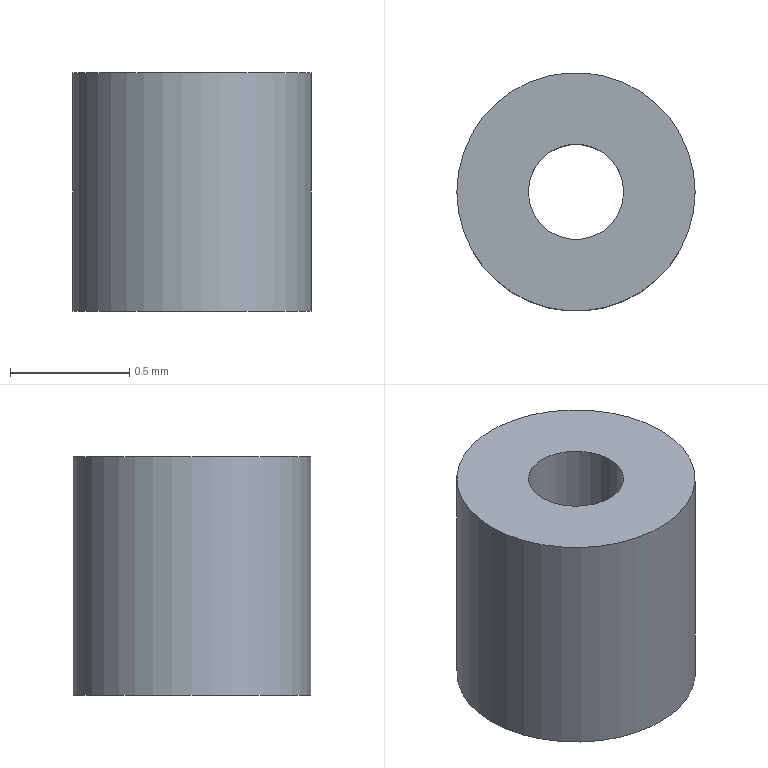Component | NX | MODEL3 | 1 solid | 4 faces | box 1 x 1 x 1 mm | volume 1 mm3 | cylinder 2 | plane 2 | commonest cylinder face diameters 1 x1 0.4 x1
STEP:
#1=CARTESIAN_POINT('',(0.,0.,0.));
#2=DIRECTION('',(0.,0.,1.));
#3=DIRECTION('',(1.,0.,0.));
#4=AXIS2_PLACEMENT_3D('',#1,#2,#3);
#5=CARTESIAN_POINT('',(69.588,-7.118,4.103));
#6=VERTEX_POINT('',#5);
#7=CARTESIAN_POINT('',(69.088,-7.118,4.103));
#8=DIRECTION('',(0.,0.,-1.));
#9=DIRECTION('',(1.,0.,0.));
#10=AXIS2_PLACEMENT_3D('',#7,#8,#9);
#11=CIRCLE('',#10,0.5);
#12=CARTESIAN_POINT('',(69.088,-7.118,4.103));
#13=DIRECTION('',(0.,0.,-1.));
#14=DIRECTION('',(-1.,0.,0.));
#15=AXIS2_PLACEMENT_3D('',#12,#13,#14);
#16=CYLINDRICAL_SURFACE('',#15,0.5);
#17=CARTESIAN_POINT('',(3.142,0.));
#18=DIRECTION('',(1.,0.));
#19=VECTOR('',#18,1.);
#20=LINE('',#17,#19);
#21=(GEOMETRIC_REPRESENTATION_CONTEXT(2)PARAMETRIC_REPRESENTATION_CONTEXT()REPRESENTATION_CONTEXT('',''));
#22=DEFINITIONAL_REPRESENTATION('',(#20),#21);
#23=PCURVE('',#16,#22);
#24=CARTESIAN_POINT('',(69.088,-7.118,4.103));
#25=DIRECTION('',(0.,0.,-1.));
#26=DIRECTION('',(-1.,0.,0.));
#27=AXIS2_PLACEMENT_3D('',#24,#25,#26);
#28=PLANE('',#27);
#29=CARTESIAN_POINT('',(0.,0.));
#30=DIRECTION('',(-1.,0.));
#31=AXIS2_PLACEMENT_2D('',#29,#30);
#32=CIRCLE('',#31,0.5);
#33=(GEOMETRIC_REPRESENTATION_CONTEXT(2)PARAMETRIC_REPRESENTATION_CONTEXT()REPRESENTATION_CONTEXT('',''));
#34=DEFINITIONAL_REPRESENTATION('',(#32),#33);
#35=PCURVE('',#28,#34);
#36=SURFACE_CURVE('',#11,(#23,#35),.PCURVE_S1.);
#37=EDGE_CURVE('',#6,#6,#36,.T.);
#38=ORIENTED_EDGE('',*,*,#37,.T.);
#39=CARTESIAN_POINT('',(69.588,-7.118,3.103));
#40=VERTEX_POINT('',#39);
#41=CARTESIAN_POINT('',(69.588,-7.118,4.103));
#42=CARTESIAN_POINT('',(69.588,-7.118,3.103));
#43=B_SPLINE_CURVE_WITH_KNOTS('',1,(#41,#42),.UNSPECIFIED.,.F.,.F.,(2,2),(0.,1.),.PIECEWISE_BEZIER_KNOTS.);
#44=CARTESIAN_POINT('',(9.425,0.));
#45=DIRECTION('',(0.,1.));
#46=VECTOR('',#45,1.);
#47=LINE('',#44,#46);
#48=(GEOMETRIC_REPRESENTATION_CONTEXT(2)PARAMETRIC_REPRESENTATION_CONTEXT()REPRESENTATION_CONTEXT('',''));
#49=DEFINITIONAL_REPRESENTATION('',(#47),#48);
#50=PCURVE('',#16,#49);
#51=CARTESIAN_POINT('',(3.142,0.));
#52=DIRECTION('',(0.,1.));
#53=VECTOR('',#52,1.);
#54=LINE('',#51,#53);
#55=(GEOMETRIC_REPRESENTATION_CONTEXT(2)PARAMETRIC_REPRESENTATION_CONTEXT()REPRESENTATION_CONTEXT('',''));
#56=DEFINITIONAL_REPRESENTATION('',(#54),#55);
#57=PCURVE('',#16,#56);
#58=SEAM_CURVE('',#43,(#50,#57),.PCURVE_S1.);
#59=EDGE_CURVE('',#6,#40,#58,.T.);
#60=ORIENTED_EDGE('',*,*,#59,.T.);
#61=CARTESIAN_POINT('',(69.088,-7.118,3.103));
#62=DIRECTION('',(0.,0.,-1.));
#63=DIRECTION('',(1.,0.,0.));
#64=AXIS2_PLACEMENT_3D('',#61,#62,#63);
#65=CIRCLE('',#64,0.5);
#66=CARTESIAN_POINT('',(3.142,1.));
#67=DIRECTION('',(1.,0.));
#68=VECTOR('',#67,1.);
#69=LINE('',#66,#68);
#70=(GEOMETRIC_REPRESENTATION_CONTEXT(2)PARAMETRIC_REPRESENTATION_CONTEXT()REPRESENTATION_CONTEXT('',''));
#71=DEFINITIONAL_REPRESENTATION('',(#69),#70);
#72=PCURVE('',#16,#71);
#73=CARTESIAN_POINT('',(69.088,-7.118,3.103));
#74=DIRECTION('',(0.,0.,-1.));
#75=DIRECTION('',(-1.,0.,0.));
#76=AXIS2_PLACEMENT_3D('',#73,#74,#75);
#77=PLANE('',#76);
#78=CARTESIAN_POINT('',(0.,0.));
#79=DIRECTION('',(-1.,0.));
#80=AXIS2_PLACEMENT_2D('',#78,#79);
#81=CIRCLE('',#80,0.5);
#82=(GEOMETRIC_REPRESENTATION_CONTEXT(2)PARAMETRIC_REPRESENTATION_CONTEXT()REPRESENTATION_CONTEXT('',''));
#83=DEFINITIONAL_REPRESENTATION('',(#81),#82);
#84=PCURVE('',#77,#83);
#85=SURFACE_CURVE('',#65,(#72,#84),.PCURVE_S1.);
#86=EDGE_CURVE('',#40,#40,#85,.T.);
#87=ORIENTED_EDGE('',*,*,#86,.F.);
#88=ORIENTED_EDGE('',*,*,#59,.F.);
#89=EDGE_LOOP('',(#38,#60,#87,#88));
#90=FACE_BOUND('',#89,.T.);
#91=ADVANCED_FACE('',(#90),#16,.T.);
#92=CARTESIAN_POINT('',(69.288,-7.118,4.103));
#93=VERTEX_POINT('',#92);
#94=CARTESIAN_POINT('',(69.088,-7.118,4.103));
#95=DIRECTION('',(0.,0.,-1.));
#96=DIRECTION('',(1.,0.,0.));
#97=AXIS2_PLACEMENT_3D('',#94,#95,#96);
#98=CIRCLE('',#97,0.2);
#99=CARTESIAN_POINT('',(69.088,-7.118,4.103));
#100=DIRECTION('',(0.,0.,-1.));
#101=DIRECTION('',(-1.,0.,0.));
#102=AXIS2_PLACEMENT_3D('',#99,#100,#101);
#103=CYLINDRICAL_SURFACE('',#102,0.2);
#104=CARTESIAN_POINT('',(3.142,0.));
#105=DIRECTION('',(1.,0.));
#106=VECTOR('',#105,1.);
#107=LINE('',#104,#106);
#108=(GEOMETRIC_REPRESENTATION_CONTEXT(2)PARAMETRIC_REPRESENTATION_CONTEXT()REPRESENTATION_CONTEXT('',''));
#109=DEFINITIONAL_REPRESENTATION('',(#107),#108);
#110=PCURVE('',#103,#109);
#111=CARTESIAN_POINT('',(0.,0.));
#112=DIRECTION('',(-1.,0.));
#113=AXIS2_PLACEMENT_2D('',#111,#112);
#114=CIRCLE('',#113,0.2);
#115=(GEOMETRIC_REPRESENTATION_CONTEXT(2)PARAMETRIC_REPRESENTATION_CONTEXT()REPRESENTATION_CONTEXT('',''));
#116=DEFINITIONAL_REPRESENTATION('',(#114),#115);
#117=PCURVE('',#28,#116);
#118=SURFACE_CURVE('',#98,(#110,#117),.PCURVE_S1.);
#119=EDGE_CURVE('',#93,#93,#118,.T.);
#120=ORIENTED_EDGE('',*,*,#119,.T.);
#121=CARTESIAN_POINT('',(69.288,-7.118,3.103));
#122=VERTEX_POINT('',#121);
#123=CARTESIAN_POINT('',(69.288,-7.118,4.103));
#124=CARTESIAN_POINT('',(69.288,-7.118,3.103));
#125=B_SPLINE_CURVE_WITH_KNOTS('',1,(#123,#124),.UNSPECIFIED.,.F.,.F.,(2,2),(0.,1.),.PIECEWISE_BEZIER_KNOTS.);
#126=CARTESIAN_POINT('',(9.425,0.));
#127=DIRECTION('',(0.,1.));
#128=VECTOR('',#127,1.);
#129=LINE('',#126,#128);
#130=(GEOMETRIC_REPRESENTATION_CONTEXT(2)PARAMETRIC_REPRESENTATION_CONTEXT()REPRESENTATION_CONTEXT('',''));
#131=DEFINITIONAL_REPRESENTATION('',(#129),#130);
#132=PCURVE('',#103,#131);
#133=CARTESIAN_POINT('',(3.142,0.));
#134=DIRECTION('',(0.,1.));
#135=VECTOR('',#134,1.);
#136=LINE('',#133,#135);
#137=(GEOMETRIC_REPRESENTATION_CONTEXT(2)PARAMETRIC_REPRESENTATION_CONTEXT()REPRESENTATION_CONTEXT('',''));
#138=DEFINITIONAL_REPRESENTATION('',(#136),#137);
#139=PCURVE('',#103,#138);
#140=SEAM_CURVE('',#125,(#132,#139),.PCURVE_S1.);
#141=EDGE_CURVE('',#93,#122,#140,.T.);
#142=ORIENTED_EDGE('',*,*,#141,.T.);
#143=CARTESIAN_POINT('',(69.088,-7.118,3.103));
#144=DIRECTION('',(0.,0.,-1.));
#145=DIRECTION('',(1.,0.,0.));
#146=AXIS2_PLACEMENT_3D('',#143,#144,#145);
#147=CIRCLE('',#146,0.2);
#148=CARTESIAN_POINT('',(3.142,1.));
#149=DIRECTION('',(1.,0.));
#150=VECTOR('',#149,1.);
#151=LINE('',#148,#150);
#152=(GEOMETRIC_REPRESENTATION_CONTEXT(2)PARAMETRIC_REPRESENTATION_CONTEXT()REPRESENTATION_CONTEXT('',''));
#153=DEFINITIONAL_REPRESENTATION('',(#151),#152);
#154=PCURVE('',#103,#153);
#155=CARTESIAN_POINT('',(0.,0.));
#156=DIRECTION('',(-1.,0.));
#157=AXIS2_PLACEMENT_2D('',#155,#156);
#158=CIRCLE('',#157,0.2);
#159=(GEOMETRIC_REPRESENTATION_CONTEXT(2)PARAMETRIC_REPRESENTATION_CONTEXT()REPRESENTATION_CONTEXT('',''));
#160=DEFINITIONAL_REPRESENTATION('',(#158),#159);
#161=PCURVE('',#77,#160);
#162=SURFACE_CURVE('',#147,(#154,#161),.PCURVE_S1.);
#163=EDGE_CURVE('',#122,#122,#162,.T.);
#164=ORIENTED_EDGE('',*,*,#163,.F.);
#165=ORIENTED_EDGE('',*,*,#141,.F.);
#166=EDGE_LOOP('',(#120,#142,#164,#165));
#167=FACE_BOUND('',#166,.F.);
#168=ADVANCED_FACE('',(#167),#103,.F.);
#169=ORIENTED_EDGE('',*,*,#37,.F.);
#170=EDGE_LOOP('',(#169));
#171=FACE_BOUND('',#170,.T.);
#172=ORIENTED_EDGE('',*,*,#119,.T.);
#173=EDGE_LOOP('',(#172));
#174=FACE_BOUND('',#173,.T.);
#175=ADVANCED_FACE('',(#171,#174),#28,.F.);
#176=ORIENTED_EDGE('',*,*,#86,.T.);
#177=EDGE_LOOP('',(#176));
#178=FACE_BOUND('',#177,.T.);
#179=ORIENTED_EDGE('',*,*,#163,.F.);
#180=EDGE_LOOP('',(#179));
#181=FACE_BOUND('',#180,.T.);
#182=ADVANCED_FACE('',(#178,#181),#77,.T.);
#183=CLOSED_SHELL('',(#91,#168,#175,#182));
#184=MANIFOLD_SOLID_BREP('',#183);
#185=(LENGTH_UNIT()NAMED_UNIT(*)SI_UNIT(.MILLI.,.METRE.));
#186=UNCERTAINTY_MEASURE_WITH_UNIT(LENGTH_MEASURE(0.00001),#185,'','');
#187=(NAMED_UNIT(*)PLANE_ANGLE_UNIT()SI_UNIT($,.RADIAN.));
#188=(NAMED_UNIT(*)SI_UNIT($,.STERADIAN.)SOLID_ANGLE_UNIT());
#189=(GEOMETRIC_REPRESENTATION_CONTEXT(3)GLOBAL_UNCERTAINTY_ASSIGNED_CONTEXT((#186))GLOBAL_UNIT_ASSIGNED_CONTEXT((#185,#187,#188))REPRESENTATION_CONTEXT('',''));
#190=ADVANCED_BREP_SHAPE_REPRESENTATION('',(#4,#184),#189);